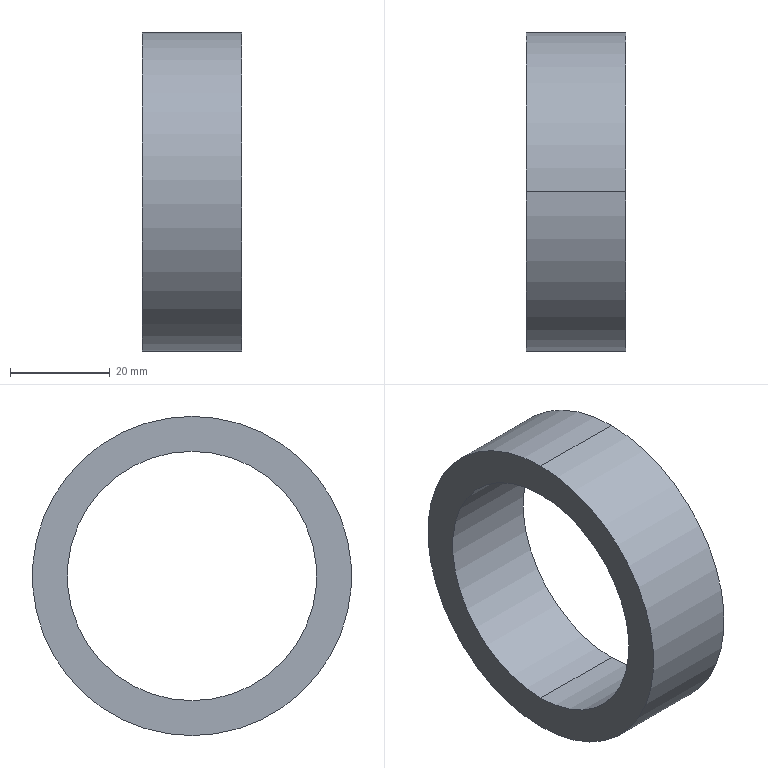Component | SolidWorks | Sleeve-1 | 1 solid | 6 faces | box 20 x 64 x 64 mm | volume 25070 mm3 | cylinder 4 | plane 2 | commonest cylinder face diameters 50 x2 64 x2
build123d program:
from build123d import *

# Parameters (mm, degrees)
SKETCH1_R           = 32
SKETCH1_R_2         = 25
BOSS_EXTRUDE1_DEPTH = 20


with BuildPart() as part:
    # Sketch1 → Boss-Extrude1 (new body)
    with BuildSketch(Plane(origin=(0, 0, 0), x_dir=(0, 0, -1), z_dir=(1, 0, 0))):
        Circle(SKETCH1_R)
        Circle(SKETCH1_R_2, mode=Mode.SUBTRACT)
    extrude(amount=BOSS_EXTRUDE1_DEPTH)


solid = part.part

# Placed as in the assembly
solid = solid.moved(Location((739.528, 15.31, -110), (0, 0, 0)))
STEP:
#1=COLOUR_RGB('',0.7922,0.8196,0.9333);
#2=FILL_AREA_STYLE_COLOUR('',#1);
#3=FILL_AREA_STYLE('',(#2));
#4=SURFACE_STYLE_FILL_AREA(#3);
#5=SURFACE_SIDE_STYLE('',(#4));
#6=SURFACE_STYLE_USAGE(.BOTH.,#5);
#7=PRESENTATION_STYLE_ASSIGNMENT((#6));
#8=CARTESIAN_POINT('',(29.903,0.6028,-3.346));
#9=VERTEX_POINT('',#8);
#10=CARTESIAN_POINT('',(29.903,0.6028,-5.315));
#11=VERTEX_POINT('',#10);
#12=CARTESIAN_POINT('',(29.903,0.6028,-4.331));
#13=DIRECTION('',(1.,0.,0.));
#14=DIRECTION('',(0.,0.,-1.));
#15=AXIS2_PLACEMENT_3D('',#12,#13,#14);
#16=CIRCLE('',#15,0.9843);
#17=EDGE_CURVE('',#9,#11,#16,.T.);
#18=ORIENTED_EDGE('',*,*,#17,.T.);
#19=CARTESIAN_POINT('',(29.115,0.6028,-5.315));
#20=VERTEX_POINT('',#19);
#21=CARTESIAN_POINT('',(29.903,0.6028,-5.315));
#22=DIRECTION('',(-1.,0.,0.));
#23=VECTOR('',#22,39.37);
#24=LINE('',#21,#23);
#25=EDGE_CURVE('',#11,#20,#24,.T.);
#26=ORIENTED_EDGE('',*,*,#25,.T.);
#27=CARTESIAN_POINT('',(29.115,0.6028,-3.346));
#28=VERTEX_POINT('',#27);
#29=CARTESIAN_POINT('',(29.115,0.6028,-4.331));
#30=DIRECTION('',(1.,0.,0.));
#31=DIRECTION('',(0.,0.,-1.));
#32=AXIS2_PLACEMENT_3D('',#29,#30,#31);
#33=CIRCLE('',#32,0.9843);
#34=EDGE_CURVE('',#28,#20,#33,.T.);
#35=ORIENTED_EDGE('',*,*,#34,.F.);
#36=CARTESIAN_POINT('',(29.903,0.6028,-3.346));
#37=DIRECTION('',(-1.,0.,0.));
#38=VECTOR('',#37,39.37);
#39=LINE('',#36,#38);
#40=EDGE_CURVE('',#9,#28,#39,.T.);
#41=ORIENTED_EDGE('',*,*,#40,.F.);
#42=EDGE_LOOP('',(#18,#26,#35,#41));
#43=FACE_OUTER_BOUND('',#42,.T.);
#44=CARTESIAN_POINT('',(29.903,0.6028,-4.331));
#45=DIRECTION('',(-1.,0.,0.));
#46=DIRECTION('',(0.,0.,1.));
#47=AXIS2_PLACEMENT_3D('',#44,#45,#46);
#48=CYLINDRICAL_SURFACE('',#47,0.9843);
#49=ADVANCED_FACE('',(#43),#48,.F.);
#50=CARTESIAN_POINT('',(29.903,0.6028,-5.591));
#51=VERTEX_POINT('',#50);
#52=CARTESIAN_POINT('',(29.903,0.6028,-3.071));
#53=VERTEX_POINT('',#52);
#54=CARTESIAN_POINT('',(29.903,0.6028,-4.331));
#55=DIRECTION('',(1.,0.,0.));
#56=DIRECTION('',(0.,0.,-1.));
#57=AXIS2_PLACEMENT_3D('',#54,#55,#56);
#58=CIRCLE('',#57,1.26);
#59=EDGE_CURVE('',#51,#53,#58,.T.);
#60=ORIENTED_EDGE('',*,*,#59,.F.);
#61=CARTESIAN_POINT('',(29.115,0.6028,-5.591));
#62=VERTEX_POINT('',#61);
#63=CARTESIAN_POINT('',(29.903,0.6028,-5.591));
#64=DIRECTION('',(-1.,0.,0.));
#65=VECTOR('',#64,39.37);
#66=LINE('',#63,#65);
#67=EDGE_CURVE('',#51,#62,#66,.T.);
#68=ORIENTED_EDGE('',*,*,#67,.T.);
#69=CARTESIAN_POINT('',(29.115,0.6028,-3.071));
#70=VERTEX_POINT('',#69);
#71=CARTESIAN_POINT('',(29.115,0.6028,-4.331));
#72=DIRECTION('',(1.,0.,0.));
#73=DIRECTION('',(0.,0.,-1.));
#74=AXIS2_PLACEMENT_3D('',#71,#72,#73);
#75=CIRCLE('',#74,1.26);
#76=EDGE_CURVE('',#62,#70,#75,.T.);
#77=ORIENTED_EDGE('',*,*,#76,.T.);
#78=CARTESIAN_POINT('',(29.903,0.6028,-3.071));
#79=DIRECTION('',(-1.,0.,0.));
#80=VECTOR('',#79,39.37);
#81=LINE('',#78,#80);
#82=EDGE_CURVE('',#53,#70,#81,.T.);
#83=ORIENTED_EDGE('',*,*,#82,.F.);
#84=EDGE_LOOP('',(#60,#68,#77,#83));
#85=FACE_OUTER_BOUND('',#84,.T.);
#86=CARTESIAN_POINT('',(29.903,0.6028,-4.331));
#87=DIRECTION('',(-1.,0.,0.));
#88=DIRECTION('',(0.,0.,1.));
#89=AXIS2_PLACEMENT_3D('',#86,#87,#88);
#90=CYLINDRICAL_SURFACE('',#89,1.26);
#91=ADVANCED_FACE('',(#85),#90,.T.);
#92=CARTESIAN_POINT('',(29.903,0.6028,-4.331));
#93=DIRECTION('',(1.,0.,0.));
#94=DIRECTION('',(0.,0.,-1.));
#95=AXIS2_PLACEMENT_3D('',#92,#93,#94);
#96=CIRCLE('',#95,1.26);
#97=EDGE_CURVE('',#53,#51,#96,.T.);
#98=ORIENTED_EDGE('',*,*,#97,.T.);
#99=ORIENTED_EDGE('',*,*,#59,.T.);
#100=EDGE_LOOP('',(#98,#99));
#101=FACE_OUTER_BOUND('',#100,.T.);
#102=ORIENTED_EDGE('',*,*,#17,.F.);
#103=CARTESIAN_POINT('',(29.903,0.6028,-4.331));
#104=DIRECTION('',(1.,0.,0.));
#105=DIRECTION('',(0.,0.,-1.));
#106=AXIS2_PLACEMENT_3D('',#103,#104,#105);
#107=CIRCLE('',#106,0.9843);
#108=EDGE_CURVE('',#11,#9,#107,.T.);
#109=ORIENTED_EDGE('',*,*,#108,.F.);
#110=EDGE_LOOP('',(#102,#109));
#111=FACE_BOUND('',#110,.T.);
#112=CARTESIAN_POINT('',(29.903,0.6028,-4.331));
#113=DIRECTION('',(1.,0.,0.));
#114=DIRECTION('',(0.,0.,-1.));
#115=AXIS2_PLACEMENT_3D('',#112,#113,#114);
#116=PLANE('',#115);
#117=ADVANCED_FACE('',(#101,#111),#116,.T.);
#118=CARTESIAN_POINT('',(29.115,0.6028,-4.331));
#119=DIRECTION('',(1.,0.,0.));
#120=DIRECTION('',(0.,0.,-1.));
#121=AXIS2_PLACEMENT_3D('',#118,#119,#120);
#122=CIRCLE('',#121,1.26);
#123=EDGE_CURVE('',#70,#62,#122,.T.);
#124=ORIENTED_EDGE('',*,*,#123,.F.);
#125=ORIENTED_EDGE('',*,*,#76,.F.);
#126=EDGE_LOOP('',(#124,#125));
#127=FACE_OUTER_BOUND('',#126,.T.);
#128=ORIENTED_EDGE('',*,*,#34,.T.);
#129=CARTESIAN_POINT('',(29.115,0.6028,-4.331));
#130=DIRECTION('',(1.,0.,0.));
#131=DIRECTION('',(0.,0.,-1.));
#132=AXIS2_PLACEMENT_3D('',#129,#130,#131);
#133=CIRCLE('',#132,0.9843);
#134=EDGE_CURVE('',#20,#28,#133,.T.);
#135=ORIENTED_EDGE('',*,*,#134,.T.);
#136=EDGE_LOOP('',(#128,#135));
#137=FACE_BOUND('',#136,.T.);
#138=CARTESIAN_POINT('',(29.115,0.6028,-4.331));
#139=DIRECTION('',(1.,0.,0.));
#140=DIRECTION('',(0.,0.,-1.));
#141=AXIS2_PLACEMENT_3D('',#138,#139,#140);
#142=PLANE('',#141);
#143=ADVANCED_FACE('',(#127,#137),#142,.F.);
#144=ORIENTED_EDGE('',*,*,#67,.F.);
#145=ORIENTED_EDGE('',*,*,#97,.F.);
#146=ORIENTED_EDGE('',*,*,#82,.T.);
#147=ORIENTED_EDGE('',*,*,#123,.T.);
#148=EDGE_LOOP('',(#144,#145,#146,#147));
#149=FACE_OUTER_BOUND('',#148,.T.);
#150=CARTESIAN_POINT('',(29.903,0.6028,-4.331));
#151=DIRECTION('',(-1.,0.,0.));
#152=DIRECTION('',(0.,0.,1.));
#153=AXIS2_PLACEMENT_3D('',#150,#151,#152);
#154=CYLINDRICAL_SURFACE('',#153,1.26);
#155=ADVANCED_FACE('',(#149),#154,.T.);
#156=ORIENTED_EDGE('',*,*,#25,.F.);
#157=ORIENTED_EDGE('',*,*,#108,.T.);
#158=ORIENTED_EDGE('',*,*,#40,.T.);
#159=ORIENTED_EDGE('',*,*,#134,.F.);
#160=EDGE_LOOP('',(#156,#157,#158,#159));
#161=FACE_OUTER_BOUND('',#160,.T.);
#162=CARTESIAN_POINT('',(29.903,0.6028,-4.331));
#163=DIRECTION('',(-1.,0.,0.));
#164=DIRECTION('',(0.,0.,1.));
#165=AXIS2_PLACEMENT_3D('',#162,#163,#164);
#166=CYLINDRICAL_SURFACE('',#165,0.9843);
#167=ADVANCED_FACE('',(#161),#166,.F.);
#168=CLOSED_SHELL('',(#49,#91,#117,#143,#155,#167));
#169=MANIFOLD_SOLID_BREP('',#168);
#170=STYLED_ITEM('',(#7),#169);
#171=PRESENTATION_LAYER_ASSIGNMENT('','',(#170));
#172=CARTESIAN_POINT('',(0.,0.,0.));
#173=DIRECTION('',(0.,0.,1.));
#174=DIRECTION('',(1.,0.,0.));
#175=AXIS2_PLACEMENT_3D('',#172,#173,#174);
#176=(LENGTH_UNIT()NAMED_UNIT(*)SI_UNIT($,.METRE.));
#177=LENGTH_MEASURE_WITH_UNIT(LENGTH_MEASURE(0.0254),#176);
#178=DIMENSIONAL_EXPONENTS(1.,0.,0.,0.,0.,0.,0.);
#179=(CONVERSION_BASED_UNIT('',#177)LENGTH_UNIT()NAMED_UNIT(#178));
#180=UNCERTAINTY_MEASURE_WITH_UNIT(LENGTH_MEASURE(0.00001),#179,'','');
#181=(NAMED_UNIT(*)PLANE_ANGLE_UNIT()SI_UNIT($,.RADIAN.));
#182=(NAMED_UNIT(*)SI_UNIT($,.STERADIAN.)SOLID_ANGLE_UNIT());
#183=(GEOMETRIC_REPRESENTATION_CONTEXT(3)GLOBAL_UNCERTAINTY_ASSIGNED_CONTEXT((#180))GLOBAL_UNIT_ASSIGNED_CONTEXT((#179,#181,#182))REPRESENTATION_CONTEXT('',''));
#184=ADVANCED_BREP_SHAPE_REPRESENTATION('',(#169,#175),#183);
#185=(LENGTH_UNIT()NAMED_UNIT(*)SI_UNIT($,.METRE.));
#186=LENGTH_MEASURE_WITH_UNIT(LENGTH_MEASURE(0.0254),#185);
#187=DIMENSIONAL_EXPONENTS(1.,0.,0.,0.,0.,0.,0.);
#188=(CONVERSION_BASED_UNIT('',#186)LENGTH_UNIT()NAMED_UNIT(#187));
#189=UNCERTAINTY_MEASURE_WITH_UNIT(LENGTH_MEASURE(0.00001),#188,'','');
#190=(NAMED_UNIT(*)PLANE_ANGLE_UNIT()SI_UNIT($,.RADIAN.));
#191=(NAMED_UNIT(*)SI_UNIT($,.STERADIAN.)SOLID_ANGLE_UNIT());
#192=(GEOMETRIC_REPRESENTATION_CONTEXT(3)GLOBAL_UNCERTAINTY_ASSIGNED_CONTEXT((#189))GLOBAL_UNIT_ASSIGNED_CONTEXT((#188,#190,#191))REPRESENTATION_CONTEXT('',''));
#193=MECHANICAL_DESIGN_GEOMETRIC_PRESENTATION_REPRESENTATION('',(#170),#192);